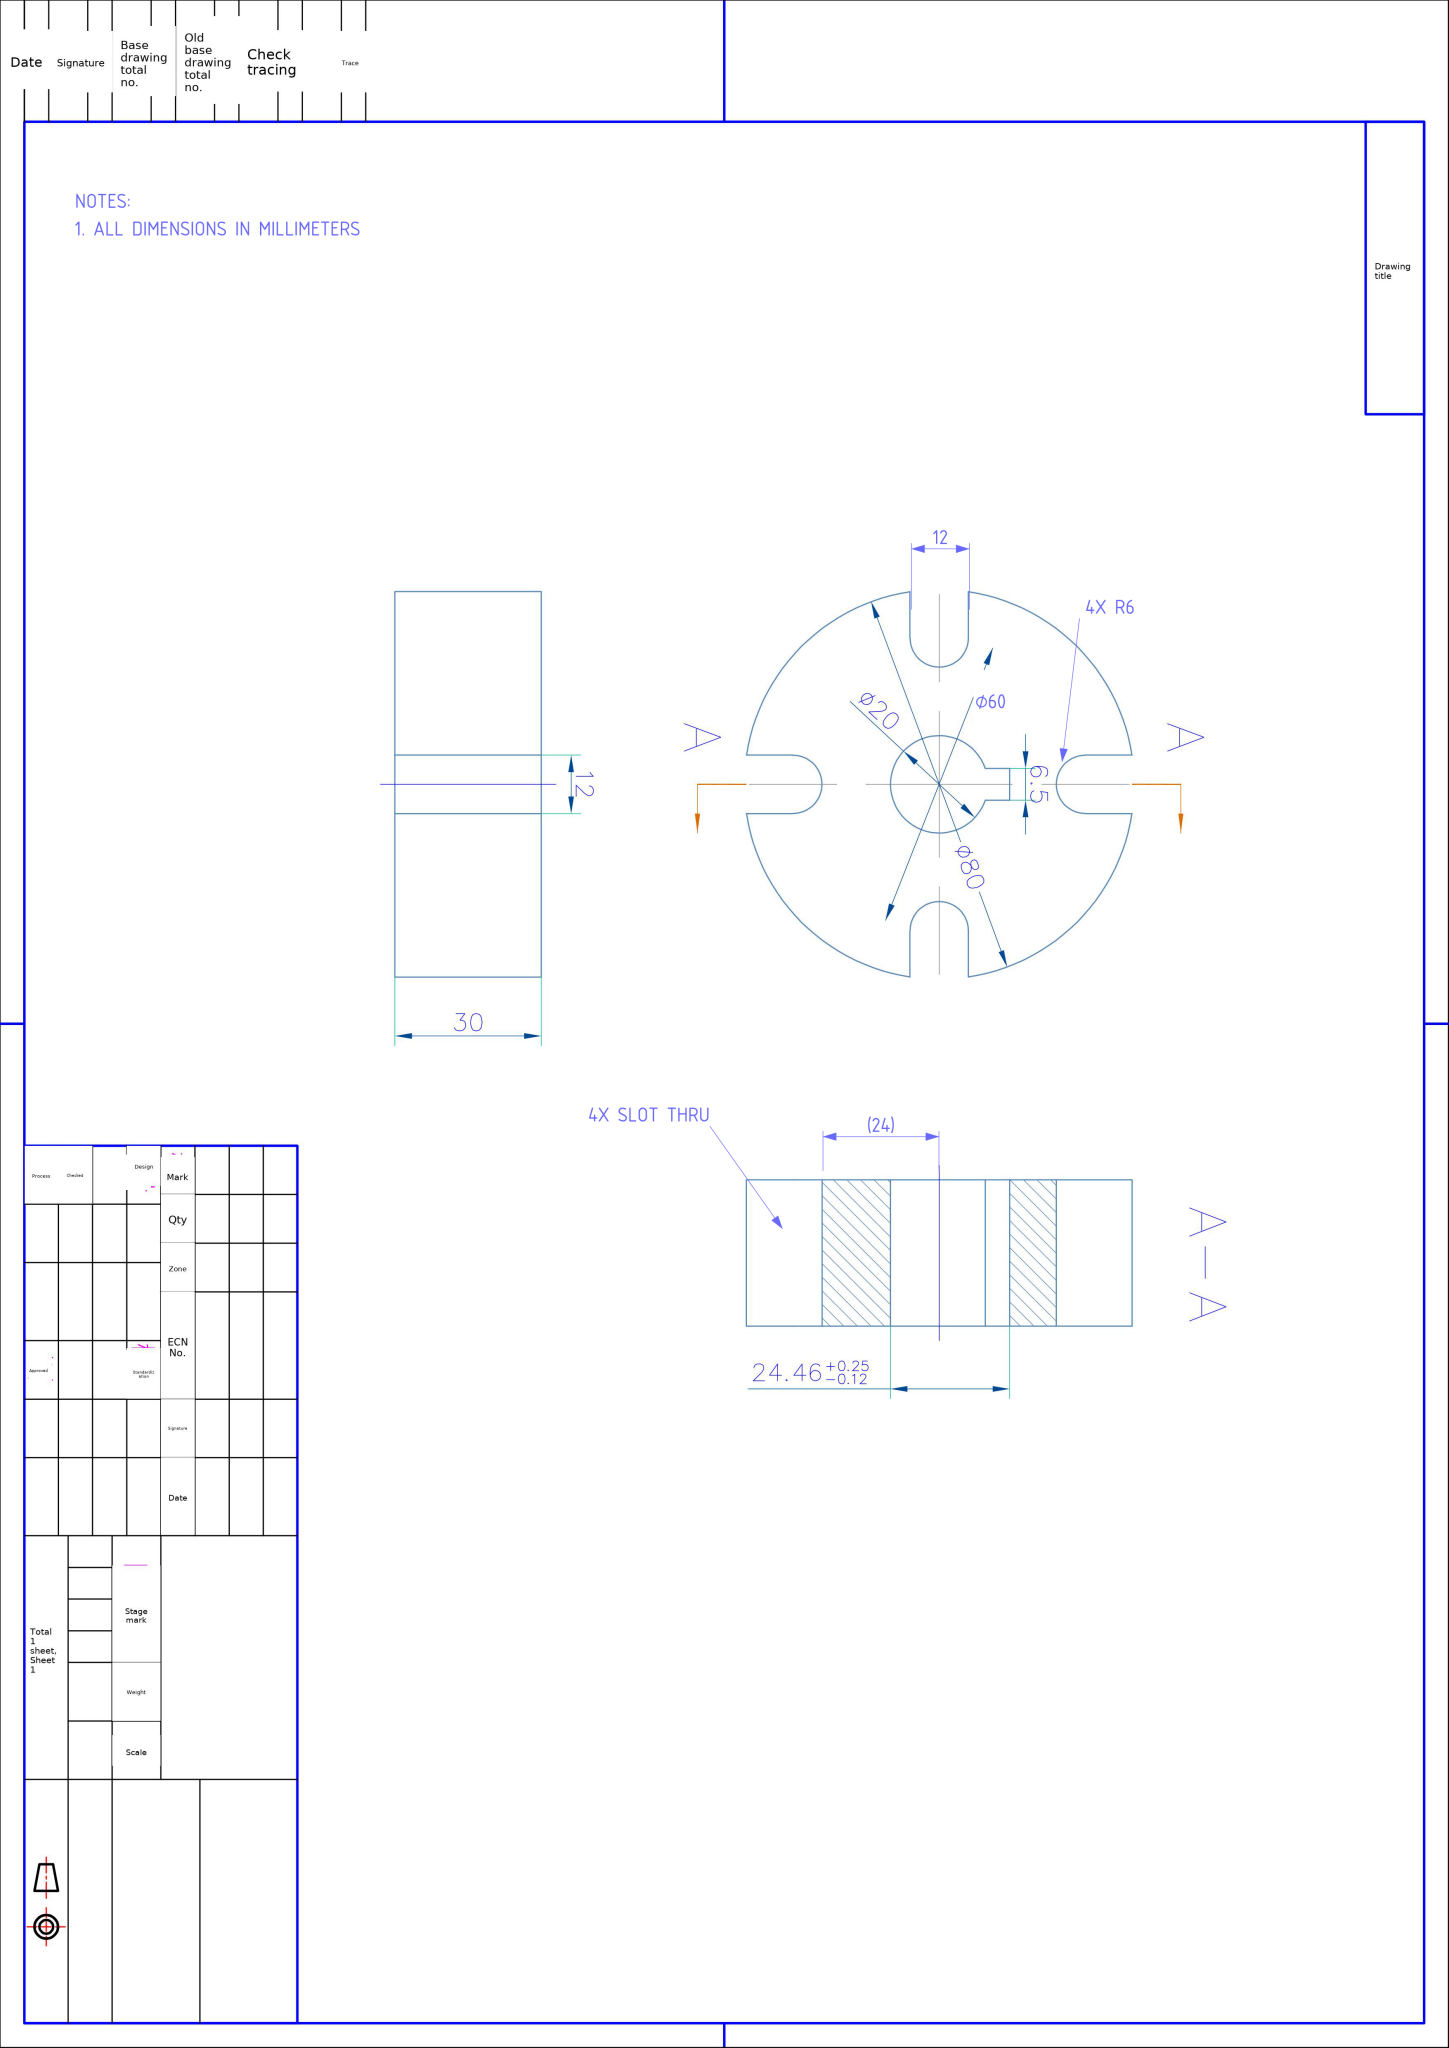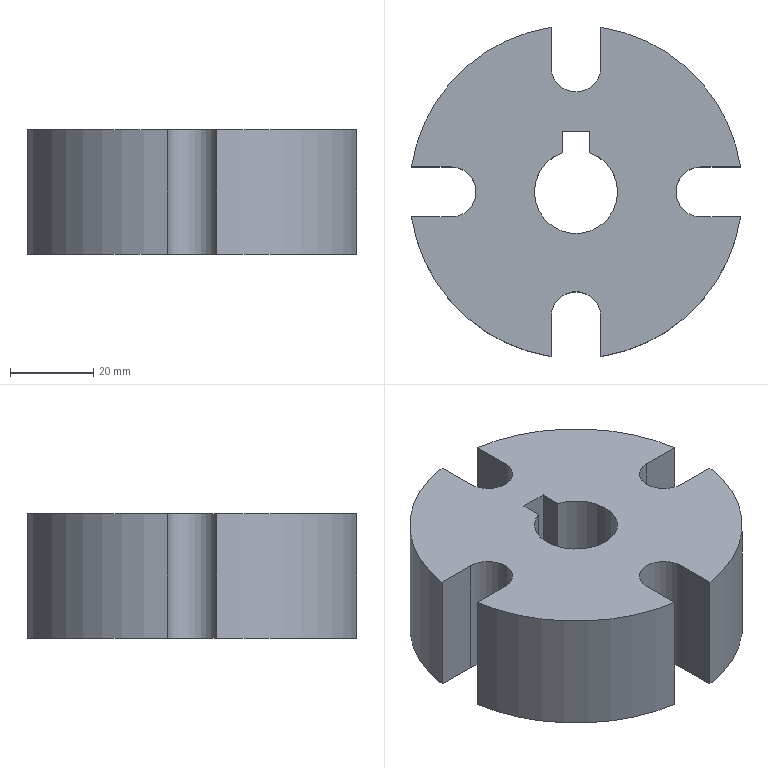Part | NX | mm | 1 solid | 22 faces | box 79.09 x 79.09 x 30 mm | volume 119499 mm3 | plane 13 | cylinder 9 | commonest cylinder face diameters 80 x4 12 x4 20 x1
STEP:
#1=CARTESIAN_POINT('',(0.,0.,0.));
#2=DIRECTION('',(0.,0.,1.));
#3=DIRECTION('',(1.,0.,0.));
#4=AXIS2_PLACEMENT_3D('',#1,#2,#3);
#5=(LENGTH_UNIT()NAMED_UNIT(*)SI_UNIT(.MILLI.,.METRE.));
#6=UNCERTAINTY_MEASURE_WITH_UNIT(LENGTH_MEASURE(0.00002),#5,'','');
#7=(NAMED_UNIT(*)PLANE_ANGLE_UNIT()SI_UNIT($,.RADIAN.));
#8=PLANE_ANGLE_MEASURE_WITH_UNIT(PLANE_ANGLE_MEASURE(0.01745),#7);
#9=DIMENSIONAL_EXPONENTS(0.,0.,0.,0.,0.,0.,0.);
#10=(CONVERSION_BASED_UNIT('',#8)NAMED_UNIT(#9)PLANE_ANGLE_UNIT());
#11=(NAMED_UNIT(*)SI_UNIT($,.STERADIAN.)SOLID_ANGLE_UNIT());
#12=(GEOMETRIC_REPRESENTATION_CONTEXT(3)GLOBAL_UNCERTAINTY_ASSIGNED_CONTEXT((#6))GLOBAL_UNIT_ASSIGNED_CONTEXT((#5,#10,#11))REPRESENTATION_CONTEXT('',''));
#13=SHAPE_REPRESENTATION('',(#4),#12);
#14=CARTESIAN_POINT('',(-3.25,9.457,0.));
#15=VERTEX_POINT('',#14);
#16=CARTESIAN_POINT('',(-3.25,14.457,0.));
#17=VERTEX_POINT('',#16);
#18=CARTESIAN_POINT('',(-3.25,9.457,0.));
#19=DIRECTION('',(0.,1.,0.));
#20=VECTOR('',#19,1.);
#21=LINE('',#18,#20);
#22=EDGE_CURVE('',#15,#17,#21,.T.);
#23=ORIENTED_EDGE('',*,*,#22,.T.);
#24=CARTESIAN_POINT('',(-3.25,14.457,30.));
#25=VERTEX_POINT('',#24);
#26=CARTESIAN_POINT('',(-3.25,14.457,30.));
#27=DIRECTION('',(0.,0.,-1.));
#28=VECTOR('',#27,1.);
#29=LINE('',#26,#28);
#30=EDGE_CURVE('',#25,#17,#29,.T.);
#31=ORIENTED_EDGE('',*,*,#30,.F.);
#32=CARTESIAN_POINT('',(-3.25,9.457,30.));
#33=VERTEX_POINT('',#32);
#34=CARTESIAN_POINT('',(-3.25,9.457,30.));
#35=DIRECTION('',(0.,1.,0.));
#36=VECTOR('',#35,1.);
#37=LINE('',#34,#36);
#38=EDGE_CURVE('',#33,#25,#37,.T.);
#39=ORIENTED_EDGE('',*,*,#38,.F.);
#40=CARTESIAN_POINT('',(-3.25,9.457,30.));
#41=DIRECTION('',(0.,0.,-1.));
#42=VECTOR('',#41,1.);
#43=LINE('',#40,#42);
#44=EDGE_CURVE('',#33,#15,#43,.T.);
#45=ORIENTED_EDGE('',*,*,#44,.T.);
#46=EDGE_LOOP('',(#23,#31,#39,#45));
#47=FACE_OUTER_BOUND('',#46,.T.);
#48=CARTESIAN_POINT('',(-3.25,9.457,30.));
#49=DIRECTION('',(-1.,0.,0.));
#50=DIRECTION('',(0.,0.,1.));
#51=AXIS2_PLACEMENT_3D('',#48,#49,#50);
#52=PLANE('',#51);
#53=ADVANCED_FACE('',(#47),#52,.F.);
#54=CARTESIAN_POINT('',(3.25,14.457,0.));
#55=VERTEX_POINT('',#54);
#56=CARTESIAN_POINT('',(-3.25,14.457,0.));
#57=DIRECTION('',(1.,0.,0.));
#58=VECTOR('',#57,1.);
#59=LINE('',#56,#58);
#60=EDGE_CURVE('',#17,#55,#59,.T.);
#61=ORIENTED_EDGE('',*,*,#60,.T.);
#62=CARTESIAN_POINT('',(3.25,14.457,30.));
#63=VERTEX_POINT('',#62);
#64=CARTESIAN_POINT('',(3.25,14.457,30.));
#65=DIRECTION('',(0.,0.,-1.));
#66=VECTOR('',#65,1.);
#67=LINE('',#64,#66);
#68=EDGE_CURVE('',#63,#55,#67,.T.);
#69=ORIENTED_EDGE('',*,*,#68,.F.);
#70=CARTESIAN_POINT('',(-3.25,14.457,30.));
#71=DIRECTION('',(1.,0.,0.));
#72=VECTOR('',#71,1.);
#73=LINE('',#70,#72);
#74=EDGE_CURVE('',#25,#63,#73,.T.);
#75=ORIENTED_EDGE('',*,*,#74,.F.);
#76=ORIENTED_EDGE('',*,*,#30,.T.);
#77=EDGE_LOOP('',(#61,#69,#75,#76));
#78=FACE_OUTER_BOUND('',#77,.T.);
#79=CARTESIAN_POINT('',(-3.25,14.457,30.));
#80=DIRECTION('',(0.,1.,0.));
#81=DIRECTION('',(0.,0.,1.));
#82=AXIS2_PLACEMENT_3D('',#79,#80,#81);
#83=PLANE('',#82);
#84=ADVANCED_FACE('',(#78),#83,.F.);
#85=CARTESIAN_POINT('',(3.25,9.457,0.));
#86=VERTEX_POINT('',#85);
#87=CARTESIAN_POINT('',(3.25,14.457,0.));
#88=DIRECTION('',(0.,-1.,0.));
#89=VECTOR('',#88,1.);
#90=LINE('',#87,#89);
#91=EDGE_CURVE('',#55,#86,#90,.T.);
#92=ORIENTED_EDGE('',*,*,#91,.T.);
#93=CARTESIAN_POINT('',(3.25,9.457,30.));
#94=VERTEX_POINT('',#93);
#95=CARTESIAN_POINT('',(3.25,9.457,30.));
#96=DIRECTION('',(0.,0.,-1.));
#97=VECTOR('',#96,1.);
#98=LINE('',#95,#97);
#99=EDGE_CURVE('',#94,#86,#98,.T.);
#100=ORIENTED_EDGE('',*,*,#99,.F.);
#101=CARTESIAN_POINT('',(3.25,14.457,30.));
#102=DIRECTION('',(0.,-1.,0.));
#103=VECTOR('',#102,1.);
#104=LINE('',#101,#103);
#105=EDGE_CURVE('',#63,#94,#104,.T.);
#106=ORIENTED_EDGE('',*,*,#105,.F.);
#107=ORIENTED_EDGE('',*,*,#68,.T.);
#108=EDGE_LOOP('',(#92,#100,#106,#107));
#109=FACE_OUTER_BOUND('',#108,.T.);
#110=CARTESIAN_POINT('',(3.25,14.457,30.));
#111=DIRECTION('',(1.,0.,0.));
#112=DIRECTION('',(0.,0.,-1.));
#113=AXIS2_PLACEMENT_3D('',#110,#111,#112);
#114=PLANE('',#113);
#115=ADVANCED_FACE('',(#109),#114,.F.);
#116=CARTESIAN_POINT('',(-30.,-6.,0.));
#117=VERTEX_POINT('',#116);
#118=CARTESIAN_POINT('',(-39.547,-6.,0.));
#119=VERTEX_POINT('',#118);
#120=CARTESIAN_POINT('',(-30.,-6.,0.));
#121=DIRECTION('',(-1.,0.,0.));
#122=VECTOR('',#121,1.);
#123=LINE('',#120,#122);
#124=EDGE_CURVE('',#117,#119,#123,.T.);
#125=ORIENTED_EDGE('',*,*,#124,.T.);
#126=CARTESIAN_POINT('',(-39.547,-6.,30.));
#127=VERTEX_POINT('',#126);
#128=CARTESIAN_POINT('',(-39.547,-6.,30.));
#129=DIRECTION('',(0.,0.,-1.));
#130=VECTOR('',#129,1.);
#131=LINE('',#128,#130);
#132=EDGE_CURVE('',#127,#119,#131,.T.);
#133=ORIENTED_EDGE('',*,*,#132,.F.);
#134=CARTESIAN_POINT('',(-30.,-6.,30.));
#135=VERTEX_POINT('',#134);
#136=CARTESIAN_POINT('',(-30.,-6.,30.));
#137=DIRECTION('',(-1.,0.,0.));
#138=VECTOR('',#137,1.);
#139=LINE('',#136,#138);
#140=EDGE_CURVE('',#135,#127,#139,.T.);
#141=ORIENTED_EDGE('',*,*,#140,.F.);
#142=CARTESIAN_POINT('',(-30.,-6.,30.));
#143=DIRECTION('',(0.,0.,-1.));
#144=VECTOR('',#143,1.);
#145=LINE('',#142,#144);
#146=EDGE_CURVE('',#135,#117,#145,.T.);
#147=ORIENTED_EDGE('',*,*,#146,.T.);
#148=EDGE_LOOP('',(#125,#133,#141,#147));
#149=FACE_OUTER_BOUND('',#148,.T.);
#150=CARTESIAN_POINT('',(-30.,-6.,30.));
#151=DIRECTION('',(-0.,-1.,0.));
#152=DIRECTION('',(1.,-0.,0.));
#153=AXIS2_PLACEMENT_3D('',#150,#151,#152);
#154=PLANE('',#153);
#155=ADVANCED_FACE('',(#149),#154,.F.);
#156=CARTESIAN_POINT('',(-6.,-39.547,0.));
#157=VERTEX_POINT('',#156);
#158=CARTESIAN_POINT('',(0.,0.,0.));
#159=DIRECTION('',(0.,0.,1.));
#160=DIRECTION('',(1.,0.,0.));
#161=AXIS2_PLACEMENT_3D('',#158,#159,#160);
#162=CIRCLE('',#161,40.);
#163=EDGE_CURVE('',#119,#157,#162,.T.);
#164=ORIENTED_EDGE('',*,*,#163,.T.);
#165=CARTESIAN_POINT('',(-6.,-39.547,30.));
#166=VERTEX_POINT('',#165);
#167=CARTESIAN_POINT('',(-6.,-39.547,30.));
#168=DIRECTION('',(0.,0.,-1.));
#169=VECTOR('',#168,1.);
#170=LINE('',#167,#169);
#171=EDGE_CURVE('',#166,#157,#170,.T.);
#172=ORIENTED_EDGE('',*,*,#171,.F.);
#173=CARTESIAN_POINT('',(0.,0.,30.));
#174=DIRECTION('',(0.,0.,1.));
#175=DIRECTION('',(1.,0.,0.));
#176=AXIS2_PLACEMENT_3D('',#173,#174,#175);
#177=CIRCLE('',#176,40.);
#178=EDGE_CURVE('',#127,#166,#177,.T.);
#179=ORIENTED_EDGE('',*,*,#178,.F.);
#180=ORIENTED_EDGE('',*,*,#132,.T.);
#181=EDGE_LOOP('',(#164,#172,#179,#180));
#182=FACE_OUTER_BOUND('',#181,.T.);
#183=CARTESIAN_POINT('',(0.,0.,30.));
#184=DIRECTION('',(0.,0.,-1.));
#185=DIRECTION('',(-1.,0.,0.));
#186=AXIS2_PLACEMENT_3D('',#183,#184,#185);
#187=CYLINDRICAL_SURFACE('',#186,40.);
#188=ADVANCED_FACE('',(#182),#187,.T.);
#189=CARTESIAN_POINT('',(-6.,-30.,0.));
#190=VERTEX_POINT('',#189);
#191=CARTESIAN_POINT('',(-6.,-39.547,0.));
#192=DIRECTION('',(0.,1.,0.));
#193=VECTOR('',#192,1.);
#194=LINE('',#191,#193);
#195=EDGE_CURVE('',#157,#190,#194,.T.);
#196=ORIENTED_EDGE('',*,*,#195,.T.);
#197=CARTESIAN_POINT('',(-6.,-30.,30.));
#198=VERTEX_POINT('',#197);
#199=CARTESIAN_POINT('',(-6.,-30.,30.));
#200=DIRECTION('',(0.,0.,-1.));
#201=VECTOR('',#200,1.);
#202=LINE('',#199,#201);
#203=EDGE_CURVE('',#198,#190,#202,.T.);
#204=ORIENTED_EDGE('',*,*,#203,.F.);
#205=CARTESIAN_POINT('',(-6.,-39.547,30.));
#206=DIRECTION('',(0.,1.,0.));
#207=VECTOR('',#206,1.);
#208=LINE('',#205,#207);
#209=EDGE_CURVE('',#166,#198,#208,.T.);
#210=ORIENTED_EDGE('',*,*,#209,.F.);
#211=ORIENTED_EDGE('',*,*,#171,.T.);
#212=EDGE_LOOP('',(#196,#204,#210,#211));
#213=FACE_OUTER_BOUND('',#212,.T.);
#214=CARTESIAN_POINT('',(-6.,-39.547,30.));
#215=DIRECTION('',(-1.,0.,0.));
#216=DIRECTION('',(-0.,-1.,0.));
#217=AXIS2_PLACEMENT_3D('',#214,#215,#216);
#218=PLANE('',#217);
#219=ADVANCED_FACE('',(#213),#218,.F.);
#220=CARTESIAN_POINT('',(6.,-30.,0.));
#221=VERTEX_POINT('',#220);
#222=CARTESIAN_POINT('',(0.,-30.,0.));
#223=DIRECTION('',(0.,0.,-1.));
#224=DIRECTION('',(1.,0.,0.));
#225=AXIS2_PLACEMENT_3D('',#222,#223,#224);
#226=CIRCLE('',#225,6.);
#227=EDGE_CURVE('',#190,#221,#226,.T.);
#228=ORIENTED_EDGE('',*,*,#227,.T.);
#229=CARTESIAN_POINT('',(6.,-30.,30.));
#230=VERTEX_POINT('',#229);
#231=CARTESIAN_POINT('',(6.,-30.,30.));
#232=DIRECTION('',(0.,0.,-1.));
#233=VECTOR('',#232,1.);
#234=LINE('',#231,#233);
#235=EDGE_CURVE('',#230,#221,#234,.T.);
#236=ORIENTED_EDGE('',*,*,#235,.F.);
#237=CARTESIAN_POINT('',(0.,-30.,30.));
#238=DIRECTION('',(0.,0.,-1.));
#239=DIRECTION('',(1.,0.,0.));
#240=AXIS2_PLACEMENT_3D('',#237,#238,#239);
#241=CIRCLE('',#240,6.);
#242=EDGE_CURVE('',#198,#230,#241,.T.);
#243=ORIENTED_EDGE('',*,*,#242,.F.);
#244=ORIENTED_EDGE('',*,*,#203,.T.);
#245=EDGE_LOOP('',(#228,#236,#243,#244));
#246=FACE_OUTER_BOUND('',#245,.T.);
#247=CARTESIAN_POINT('',(0.,-30.,30.));
#248=DIRECTION('',(0.,0.,-1.));
#249=DIRECTION('',(-1.,0.,0.));
#250=AXIS2_PLACEMENT_3D('',#247,#248,#249);
#251=CYLINDRICAL_SURFACE('',#250,6.);
#252=ADVANCED_FACE('',(#246),#251,.F.);
#253=CARTESIAN_POINT('',(6.,-39.547,0.));
#254=VERTEX_POINT('',#253);
#255=CARTESIAN_POINT('',(6.,-30.,0.));
#256=DIRECTION('',(0.,-1.,0.));
#257=VECTOR('',#256,1.);
#258=LINE('',#255,#257);
#259=EDGE_CURVE('',#221,#254,#258,.T.);
#260=ORIENTED_EDGE('',*,*,#259,.T.);
#261=CARTESIAN_POINT('',(6.,-39.547,30.));
#262=VERTEX_POINT('',#261);
#263=CARTESIAN_POINT('',(6.,-39.547,30.));
#264=DIRECTION('',(0.,0.,-1.));
#265=VECTOR('',#264,1.);
#266=LINE('',#263,#265);
#267=EDGE_CURVE('',#262,#254,#266,.T.);
#268=ORIENTED_EDGE('',*,*,#267,.F.);
#269=CARTESIAN_POINT('',(6.,-30.,30.));
#270=DIRECTION('',(0.,-1.,0.));
#271=VECTOR('',#270,1.);
#272=LINE('',#269,#271);
#273=EDGE_CURVE('',#230,#262,#272,.T.);
#274=ORIENTED_EDGE('',*,*,#273,.F.);
#275=ORIENTED_EDGE('',*,*,#235,.T.);
#276=EDGE_LOOP('',(#260,#268,#274,#275));
#277=FACE_OUTER_BOUND('',#276,.T.);
#278=CARTESIAN_POINT('',(6.,-30.,30.));
#279=DIRECTION('',(1.,0.,0.));
#280=DIRECTION('',(-0.,1.,0.));
#281=AXIS2_PLACEMENT_3D('',#278,#279,#280);
#282=PLANE('',#281);
#283=ADVANCED_FACE('',(#277),#282,.F.);
#284=CARTESIAN_POINT('',(39.547,-6.,0.));
#285=VERTEX_POINT('',#284);
#286=CARTESIAN_POINT('',(0.,0.,0.));
#287=DIRECTION('',(0.,0.,1.));
#288=DIRECTION('',(1.,0.,0.));
#289=AXIS2_PLACEMENT_3D('',#286,#287,#288);
#290=CIRCLE('',#289,40.);
#291=EDGE_CURVE('',#254,#285,#290,.T.);
#292=ORIENTED_EDGE('',*,*,#291,.T.);
#293=CARTESIAN_POINT('',(39.547,-6.,30.));
#294=VERTEX_POINT('',#293);
#295=CARTESIAN_POINT('',(39.547,-6.,30.));
#296=DIRECTION('',(0.,0.,-1.));
#297=VECTOR('',#296,1.);
#298=LINE('',#295,#297);
#299=EDGE_CURVE('',#294,#285,#298,.T.);
#300=ORIENTED_EDGE('',*,*,#299,.F.);
#301=CARTESIAN_POINT('',(0.,0.,30.));
#302=DIRECTION('',(0.,0.,1.));
#303=DIRECTION('',(1.,0.,0.));
#304=AXIS2_PLACEMENT_3D('',#301,#302,#303);
#305=CIRCLE('',#304,40.);
#306=EDGE_CURVE('',#262,#294,#305,.T.);
#307=ORIENTED_EDGE('',*,*,#306,.F.);
#308=ORIENTED_EDGE('',*,*,#267,.T.);
#309=EDGE_LOOP('',(#292,#300,#307,#308));
#310=FACE_OUTER_BOUND('',#309,.T.);
#311=CARTESIAN_POINT('',(0.,0.,30.));
#312=DIRECTION('',(0.,0.,-1.));
#313=DIRECTION('',(-1.,0.,0.));
#314=AXIS2_PLACEMENT_3D('',#311,#312,#313);
#315=CYLINDRICAL_SURFACE('',#314,40.);
#316=ADVANCED_FACE('',(#310),#315,.T.);
#317=CARTESIAN_POINT('',(30.,-6.,0.));
#318=VERTEX_POINT('',#317);
#319=CARTESIAN_POINT('',(39.547,-6.,0.));
#320=DIRECTION('',(-1.,-0.,0.));
#321=VECTOR('',#320,1.);
#322=LINE('',#319,#321);
#323=EDGE_CURVE('',#285,#318,#322,.T.);
#324=ORIENTED_EDGE('',*,*,#323,.T.);
#325=CARTESIAN_POINT('',(30.,-6.,30.));
#326=VERTEX_POINT('',#325);
#327=CARTESIAN_POINT('',(30.,-6.,30.));
#328=DIRECTION('',(0.,0.,-1.));
#329=VECTOR('',#328,1.);
#330=LINE('',#327,#329);
#331=EDGE_CURVE('',#326,#318,#330,.T.);
#332=ORIENTED_EDGE('',*,*,#331,.F.);
#333=CARTESIAN_POINT('',(39.547,-6.,30.));
#334=DIRECTION('',(-1.,-0.,0.));
#335=VECTOR('',#334,1.);
#336=LINE('',#333,#335);
#337=EDGE_CURVE('',#294,#326,#336,.T.);
#338=ORIENTED_EDGE('',*,*,#337,.F.);
#339=ORIENTED_EDGE('',*,*,#299,.T.);
#340=EDGE_LOOP('',(#324,#332,#338,#339));
#341=FACE_OUTER_BOUND('',#340,.T.);
#342=CARTESIAN_POINT('',(39.547,-6.,30.));
#343=DIRECTION('',(0.,-1.,0.));
#344=DIRECTION('',(1.,0.,0.));
#345=AXIS2_PLACEMENT_3D('',#342,#343,#344);
#346=PLANE('',#345);
#347=ADVANCED_FACE('',(#341),#346,.F.);
#348=CARTESIAN_POINT('',(30.,6.,0.));
#349=VERTEX_POINT('',#348);
#350=CARTESIAN_POINT('',(30.,0.,0.));
#351=DIRECTION('',(0.,0.,-1.));
#352=DIRECTION('',(1.,0.,0.));
#353=AXIS2_PLACEMENT_3D('',#350,#351,#352);
#354=CIRCLE('',#353,6.);
#355=EDGE_CURVE('',#318,#349,#354,.T.);
#356=ORIENTED_EDGE('',*,*,#355,.T.);
#357=CARTESIAN_POINT('',(30.,6.,30.));
#358=VERTEX_POINT('',#357);
#359=CARTESIAN_POINT('',(30.,6.,30.));
#360=DIRECTION('',(0.,0.,-1.));
#361=VECTOR('',#360,1.);
#362=LINE('',#359,#361);
#363=EDGE_CURVE('',#358,#349,#362,.T.);
#364=ORIENTED_EDGE('',*,*,#363,.F.);
#365=CARTESIAN_POINT('',(30.,0.,30.));
#366=DIRECTION('',(0.,0.,-1.));
#367=DIRECTION('',(1.,0.,0.));
#368=AXIS2_PLACEMENT_3D('',#365,#366,#367);
#369=CIRCLE('',#368,6.);
#370=EDGE_CURVE('',#326,#358,#369,.T.);
#371=ORIENTED_EDGE('',*,*,#370,.F.);
#372=ORIENTED_EDGE('',*,*,#331,.T.);
#373=EDGE_LOOP('',(#356,#364,#371,#372));
#374=FACE_OUTER_BOUND('',#373,.T.);
#375=CARTESIAN_POINT('',(30.,0.,30.));
#376=DIRECTION('',(0.,0.,-1.));
#377=DIRECTION('',(-1.,0.,0.));
#378=AXIS2_PLACEMENT_3D('',#375,#376,#377);
#379=CYLINDRICAL_SURFACE('',#378,6.);
#380=ADVANCED_FACE('',(#374),#379,.F.);
#381=CARTESIAN_POINT('',(39.547,6.,0.));
#382=VERTEX_POINT('',#381);
#383=CARTESIAN_POINT('',(30.,6.,0.));
#384=DIRECTION('',(1.,-0.,0.));
#385=VECTOR('',#384,1.);
#386=LINE('',#383,#385);
#387=EDGE_CURVE('',#349,#382,#386,.T.);
#388=ORIENTED_EDGE('',*,*,#387,.T.);
#389=CARTESIAN_POINT('',(39.547,6.,30.));
#390=VERTEX_POINT('',#389);
#391=CARTESIAN_POINT('',(39.547,6.,30.));
#392=DIRECTION('',(0.,0.,-1.));
#393=VECTOR('',#392,1.);
#394=LINE('',#391,#393);
#395=EDGE_CURVE('',#390,#382,#394,.T.);
#396=ORIENTED_EDGE('',*,*,#395,.F.);
#397=CARTESIAN_POINT('',(30.,6.,30.));
#398=DIRECTION('',(1.,-0.,0.));
#399=VECTOR('',#398,1.);
#400=LINE('',#397,#399);
#401=EDGE_CURVE('',#358,#390,#400,.T.);
#402=ORIENTED_EDGE('',*,*,#401,.F.);
#403=ORIENTED_EDGE('',*,*,#363,.T.);
#404=EDGE_LOOP('',(#388,#396,#402,#403));
#405=FACE_OUTER_BOUND('',#404,.T.);
#406=CARTESIAN_POINT('',(30.,6.,30.));
#407=DIRECTION('',(0.,1.,0.));
#408=DIRECTION('',(-1.,0.,0.));
#409=AXIS2_PLACEMENT_3D('',#406,#407,#408);
#410=PLANE('',#409);
#411=ADVANCED_FACE('',(#405),#410,.F.);
#412=CARTESIAN_POINT('',(6.,39.547,0.));
#413=VERTEX_POINT('',#412);
#414=CARTESIAN_POINT('',(0.,0.,0.));
#415=DIRECTION('',(0.,0.,1.));
#416=DIRECTION('',(1.,0.,0.));
#417=AXIS2_PLACEMENT_3D('',#414,#415,#416);
#418=CIRCLE('',#417,40.);
#419=EDGE_CURVE('',#382,#413,#418,.T.);
#420=ORIENTED_EDGE('',*,*,#419,.T.);
#421=CARTESIAN_POINT('',(6.,39.547,30.));
#422=VERTEX_POINT('',#421);
#423=CARTESIAN_POINT('',(6.,39.547,30.));
#424=DIRECTION('',(0.,0.,-1.));
#425=VECTOR('',#424,1.);
#426=LINE('',#423,#425);
#427=EDGE_CURVE('',#422,#413,#426,.T.);
#428=ORIENTED_EDGE('',*,*,#427,.F.);
#429=CARTESIAN_POINT('',(0.,0.,30.));
#430=DIRECTION('',(0.,0.,1.));
#431=DIRECTION('',(1.,0.,0.));
#432=AXIS2_PLACEMENT_3D('',#429,#430,#431);
#433=CIRCLE('',#432,40.);
#434=EDGE_CURVE('',#390,#422,#433,.T.);
#435=ORIENTED_EDGE('',*,*,#434,.F.);
#436=ORIENTED_EDGE('',*,*,#395,.T.);
#437=EDGE_LOOP('',(#420,#428,#435,#436));
#438=FACE_OUTER_BOUND('',#437,.T.);
#439=CARTESIAN_POINT('',(0.,0.,30.));
#440=DIRECTION('',(0.,0.,-1.));
#441=DIRECTION('',(-1.,0.,0.));
#442=AXIS2_PLACEMENT_3D('',#439,#440,#441);
#443=CYLINDRICAL_SURFACE('',#442,40.);
#444=ADVANCED_FACE('',(#438),#443,.T.);
#445=CARTESIAN_POINT('',(6.,30.,0.));
#446=VERTEX_POINT('',#445);
#447=CARTESIAN_POINT('',(6.,39.547,0.));
#448=DIRECTION('',(-0.,-1.,0.));
#449=VECTOR('',#448,1.);
#450=LINE('',#447,#449);
#451=EDGE_CURVE('',#413,#446,#450,.T.);
#452=ORIENTED_EDGE('',*,*,#451,.T.);
#453=CARTESIAN_POINT('',(6.,30.,30.));
#454=VERTEX_POINT('',#453);
#455=CARTESIAN_POINT('',(6.,30.,30.));
#456=DIRECTION('',(0.,0.,-1.));
#457=VECTOR('',#456,1.);
#458=LINE('',#455,#457);
#459=EDGE_CURVE('',#454,#446,#458,.T.);
#460=ORIENTED_EDGE('',*,*,#459,.F.);
#461=CARTESIAN_POINT('',(6.,39.547,30.));
#462=DIRECTION('',(-0.,-1.,0.));
#463=VECTOR('',#462,1.);
#464=LINE('',#461,#463);
#465=EDGE_CURVE('',#422,#454,#464,.T.);
#466=ORIENTED_EDGE('',*,*,#465,.F.);
#467=ORIENTED_EDGE('',*,*,#427,.T.);
#468=EDGE_LOOP('',(#452,#460,#466,#467));
#469=FACE_OUTER_BOUND('',#468,.T.);
#470=CARTESIAN_POINT('',(6.,39.547,30.));
#471=DIRECTION('',(1.,-0.,0.));
#472=DIRECTION('',(0.,1.,0.));
#473=AXIS2_PLACEMENT_3D('',#470,#471,#472);
#474=PLANE('',#473);
#475=ADVANCED_FACE('',(#469),#474,.F.);
#476=CARTESIAN_POINT('',(-6.,30.,0.));
#477=VERTEX_POINT('',#476);
#478=CARTESIAN_POINT('',(0.,30.,0.));
#479=DIRECTION('',(0.,0.,-1.));
#480=DIRECTION('',(1.,0.,0.));
#481=AXIS2_PLACEMENT_3D('',#478,#479,#480);
#482=CIRCLE('',#481,6.);
#483=EDGE_CURVE('',#446,#477,#482,.T.);
#484=ORIENTED_EDGE('',*,*,#483,.T.);
#485=CARTESIAN_POINT('',(-6.,30.,30.));
#486=VERTEX_POINT('',#485);
#487=CARTESIAN_POINT('',(-6.,30.,30.));
#488=DIRECTION('',(0.,0.,-1.));
#489=VECTOR('',#488,1.);
#490=LINE('',#487,#489);
#491=EDGE_CURVE('',#486,#477,#490,.T.);
#492=ORIENTED_EDGE('',*,*,#491,.F.);
#493=CARTESIAN_POINT('',(0.,30.,30.));
#494=DIRECTION('',(0.,0.,-1.));
#495=DIRECTION('',(1.,0.,0.));
#496=AXIS2_PLACEMENT_3D('',#493,#494,#495);
#497=CIRCLE('',#496,6.);
#498=EDGE_CURVE('',#454,#486,#497,.T.);
#499=ORIENTED_EDGE('',*,*,#498,.F.);
#500=ORIENTED_EDGE('',*,*,#459,.T.);
#501=EDGE_LOOP('',(#484,#492,#499,#500));
#502=FACE_OUTER_BOUND('',#501,.T.);
#503=CARTESIAN_POINT('',(0.,30.,30.));
#504=DIRECTION('',(0.,0.,-1.));
#505=DIRECTION('',(-1.,0.,0.));
#506=AXIS2_PLACEMENT_3D('',#503,#504,#505);
#507=CYLINDRICAL_SURFACE('',#506,6.);
#508=ADVANCED_FACE('',(#502),#507,.F.);
#509=CARTESIAN_POINT('',(-6.,39.547,0.));
#510=VERTEX_POINT('',#509);
#511=CARTESIAN_POINT('',(-6.,30.,0.));
#512=DIRECTION('',(-0.,1.,0.));
#513=VECTOR('',#512,1.);
#514=LINE('',#511,#513);
#515=EDGE_CURVE('',#477,#510,#514,.T.);
#516=ORIENTED_EDGE('',*,*,#515,.T.);
#517=CARTESIAN_POINT('',(-6.,39.547,30.));
#518=VERTEX_POINT('',#517);
#519=CARTESIAN_POINT('',(-6.,39.547,30.));
#520=DIRECTION('',(0.,0.,-1.));
#521=VECTOR('',#520,1.);
#522=LINE('',#519,#521);
#523=EDGE_CURVE('',#518,#510,#522,.T.);
#524=ORIENTED_EDGE('',*,*,#523,.F.);
#525=CARTESIAN_POINT('',(-6.,30.,30.));
#526=DIRECTION('',(-0.,1.,0.));
#527=VECTOR('',#526,1.);
#528=LINE('',#525,#527);
#529=EDGE_CURVE('',#486,#518,#528,.T.);
#530=ORIENTED_EDGE('',*,*,#529,.F.);
#531=ORIENTED_EDGE('',*,*,#491,.T.);
#532=EDGE_LOOP('',(#516,#524,#530,#531));
#533=FACE_OUTER_BOUND('',#532,.T.);
#534=CARTESIAN_POINT('',(-6.,30.,30.));
#535=DIRECTION('',(-1.,-0.,0.));
#536=DIRECTION('',(0.,-1.,0.));
#537=AXIS2_PLACEMENT_3D('',#534,#535,#536);
#538=PLANE('',#537);
#539=ADVANCED_FACE('',(#533),#538,.F.);
#540=CARTESIAN_POINT('',(-39.547,6.,0.));
#541=VERTEX_POINT('',#540);
#542=CARTESIAN_POINT('',(0.,0.,0.));
#543=DIRECTION('',(0.,0.,1.));
#544=DIRECTION('',(1.,0.,0.));
#545=AXIS2_PLACEMENT_3D('',#542,#543,#544);
#546=CIRCLE('',#545,40.);
#547=EDGE_CURVE('',#510,#541,#546,.T.);
#548=ORIENTED_EDGE('',*,*,#547,.T.);
#549=CARTESIAN_POINT('',(-39.547,6.,30.));
#550=VERTEX_POINT('',#549);
#551=CARTESIAN_POINT('',(-39.547,6.,30.));
#552=DIRECTION('',(0.,0.,-1.));
#553=VECTOR('',#552,1.);
#554=LINE('',#551,#553);
#555=EDGE_CURVE('',#550,#541,#554,.T.);
#556=ORIENTED_EDGE('',*,*,#555,.F.);
#557=CARTESIAN_POINT('',(0.,0.,30.));
#558=DIRECTION('',(0.,0.,1.));
#559=DIRECTION('',(1.,0.,0.));
#560=AXIS2_PLACEMENT_3D('',#557,#558,#559);
#561=CIRCLE('',#560,40.);
#562=EDGE_CURVE('',#518,#550,#561,.T.);
#563=ORIENTED_EDGE('',*,*,#562,.F.);
#564=ORIENTED_EDGE('',*,*,#523,.T.);
#565=EDGE_LOOP('',(#548,#556,#563,#564));
#566=FACE_OUTER_BOUND('',#565,.T.);
#567=CARTESIAN_POINT('',(0.,0.,30.));
#568=DIRECTION('',(0.,0.,-1.));
#569=DIRECTION('',(-1.,0.,0.));
#570=AXIS2_PLACEMENT_3D('',#567,#568,#569);
#571=CYLINDRICAL_SURFACE('',#570,40.);
#572=ADVANCED_FACE('',(#566),#571,.T.);
#573=CARTESIAN_POINT('',(-30.,6.,0.));
#574=VERTEX_POINT('',#573);
#575=CARTESIAN_POINT('',(-39.547,6.,0.));
#576=DIRECTION('',(1.,0.,0.));
#577=VECTOR('',#576,1.);
#578=LINE('',#575,#577);
#579=EDGE_CURVE('',#541,#574,#578,.T.);
#580=ORIENTED_EDGE('',*,*,#579,.T.);
#581=CARTESIAN_POINT('',(-30.,6.,30.));
#582=VERTEX_POINT('',#581);
#583=CARTESIAN_POINT('',(-30.,6.,30.));
#584=DIRECTION('',(0.,0.,-1.));
#585=VECTOR('',#584,1.);
#586=LINE('',#583,#585);
#587=EDGE_CURVE('',#582,#574,#586,.T.);
#588=ORIENTED_EDGE('',*,*,#587,.F.);
#589=CARTESIAN_POINT('',(-39.547,6.,30.));
#590=DIRECTION('',(1.,0.,0.));
#591=VECTOR('',#590,1.);
#592=LINE('',#589,#591);
#593=EDGE_CURVE('',#550,#582,#592,.T.);
#594=ORIENTED_EDGE('',*,*,#593,.F.);
#595=ORIENTED_EDGE('',*,*,#555,.T.);
#596=EDGE_LOOP('',(#580,#588,#594,#595));
#597=FACE_OUTER_BOUND('',#596,.T.);
#598=CARTESIAN_POINT('',(-39.547,6.,30.));
#599=DIRECTION('',(-0.,1.,0.));
#600=DIRECTION('',(-1.,-0.,0.));
#601=AXIS2_PLACEMENT_3D('',#598,#599,#600);
#602=PLANE('',#601);
#603=ADVANCED_FACE('',(#597),#602,.F.);
#604=CARTESIAN_POINT('',(-30.,0.,0.));
#605=DIRECTION('',(0.,0.,-1.));
#606=DIRECTION('',(1.,0.,0.));
#607=AXIS2_PLACEMENT_3D('',#604,#605,#606);
#608=CIRCLE('',#607,6.);
#609=EDGE_CURVE('',#574,#117,#608,.T.);
#610=ORIENTED_EDGE('',*,*,#609,.T.);
#611=ORIENTED_EDGE('',*,*,#146,.F.);
#612=CARTESIAN_POINT('',(-30.,0.,30.));
#613=DIRECTION('',(0.,0.,-1.));
#614=DIRECTION('',(1.,0.,0.));
#615=AXIS2_PLACEMENT_3D('',#612,#613,#614);
#616=CIRCLE('',#615,6.);
#617=EDGE_CURVE('',#582,#135,#616,.T.);
#618=ORIENTED_EDGE('',*,*,#617,.F.);
#619=ORIENTED_EDGE('',*,*,#587,.T.);
#620=EDGE_LOOP('',(#610,#611,#618,#619));
#621=FACE_OUTER_BOUND('',#620,.T.);
#622=CARTESIAN_POINT('',(-30.,0.,30.));
#623=DIRECTION('',(0.,0.,-1.));
#624=DIRECTION('',(-1.,0.,0.));
#625=AXIS2_PLACEMENT_3D('',#622,#623,#624);
#626=CYLINDRICAL_SURFACE('',#625,6.);
#627=ADVANCED_FACE('',(#621),#626,.F.);
#628=CARTESIAN_POINT('',(0.,0.,0.));
#629=DIRECTION('',(0.,0.,-1.));
#630=DIRECTION('',(1.,0.,0.));
#631=AXIS2_PLACEMENT_3D('',#628,#629,#630);
#632=CIRCLE('',#631,10.);
#633=EDGE_CURVE('',#86,#15,#632,.T.);
#634=ORIENTED_EDGE('',*,*,#633,.T.);
#635=ORIENTED_EDGE('',*,*,#44,.F.);
#636=CARTESIAN_POINT('',(0.,0.,30.));
#637=DIRECTION('',(0.,0.,-1.));
#638=DIRECTION('',(1.,0.,0.));
#639=AXIS2_PLACEMENT_3D('',#636,#637,#638);
#640=CIRCLE('',#639,10.);
#641=EDGE_CURVE('',#94,#33,#640,.T.);
#642=ORIENTED_EDGE('',*,*,#641,.F.);
#643=ORIENTED_EDGE('',*,*,#99,.T.);
#644=EDGE_LOOP('',(#634,#635,#642,#643));
#645=FACE_OUTER_BOUND('',#644,.T.);
#646=CARTESIAN_POINT('',(0.,0.,30.));
#647=DIRECTION('',(0.,0.,-1.));
#648=DIRECTION('',(-1.,0.,0.));
#649=AXIS2_PLACEMENT_3D('',#646,#647,#648);
#650=CYLINDRICAL_SURFACE('',#649,10.);
#651=ADVANCED_FACE('',(#645),#650,.F.);
#652=ORIENTED_EDGE('',*,*,#140,.T.);
#653=ORIENTED_EDGE('',*,*,#178,.T.);
#654=ORIENTED_EDGE('',*,*,#209,.T.);
#655=ORIENTED_EDGE('',*,*,#242,.T.);
#656=ORIENTED_EDGE('',*,*,#273,.T.);
#657=ORIENTED_EDGE('',*,*,#306,.T.);
#658=ORIENTED_EDGE('',*,*,#337,.T.);
#659=ORIENTED_EDGE('',*,*,#370,.T.);
#660=ORIENTED_EDGE('',*,*,#401,.T.);
#661=ORIENTED_EDGE('',*,*,#434,.T.);
#662=ORIENTED_EDGE('',*,*,#465,.T.);
#663=ORIENTED_EDGE('',*,*,#498,.T.);
#664=ORIENTED_EDGE('',*,*,#529,.T.);
#665=ORIENTED_EDGE('',*,*,#562,.T.);
#666=ORIENTED_EDGE('',*,*,#593,.T.);
#667=ORIENTED_EDGE('',*,*,#617,.T.);
#668=EDGE_LOOP('',(#652,#653,#654,#655,#656,#657,#658,#659,#660,#661,#662,#663,#664,#665,#666,#667));
#669=FACE_BOUND('',#668,.T.);
#670=ORIENTED_EDGE('',*,*,#38,.T.);
#671=ORIENTED_EDGE('',*,*,#74,.T.);
#672=ORIENTED_EDGE('',*,*,#105,.T.);
#673=ORIENTED_EDGE('',*,*,#641,.T.);
#674=EDGE_LOOP('',(#670,#671,#672,#673));
#675=FACE_BOUND('',#674,.T.);
#676=CARTESIAN_POINT('',(0.,0.,30.));
#677=DIRECTION('',(0.,0.,1.));
#678=DIRECTION('',(1.,0.,0.));
#679=AXIS2_PLACEMENT_3D('',#676,#677,#678);
#680=PLANE('',#679);
#681=ADVANCED_FACE('',(#669,#675),#680,.T.);
#682=ORIENTED_EDGE('',*,*,#124,.F.);
#683=ORIENTED_EDGE('',*,*,#609,.F.);
#684=ORIENTED_EDGE('',*,*,#579,.F.);
#685=ORIENTED_EDGE('',*,*,#547,.F.);
#686=ORIENTED_EDGE('',*,*,#515,.F.);
#687=ORIENTED_EDGE('',*,*,#483,.F.);
#688=ORIENTED_EDGE('',*,*,#451,.F.);
#689=ORIENTED_EDGE('',*,*,#419,.F.);
#690=ORIENTED_EDGE('',*,*,#387,.F.);
#691=ORIENTED_EDGE('',*,*,#355,.F.);
#692=ORIENTED_EDGE('',*,*,#323,.F.);
#693=ORIENTED_EDGE('',*,*,#291,.F.);
#694=ORIENTED_EDGE('',*,*,#259,.F.);
#695=ORIENTED_EDGE('',*,*,#227,.F.);
#696=ORIENTED_EDGE('',*,*,#195,.F.);
#697=ORIENTED_EDGE('',*,*,#163,.F.);
#698=EDGE_LOOP('',(#682,#683,#684,#685,#686,#687,#688,#689,#690,#691,#692,#693,#694,#695,#696,#697));
#699=FACE_BOUND('',#698,.T.);
#700=ORIENTED_EDGE('',*,*,#22,.F.);
#701=ORIENTED_EDGE('',*,*,#633,.F.);
#702=ORIENTED_EDGE('',*,*,#91,.F.);
#703=ORIENTED_EDGE('',*,*,#60,.F.);
#704=EDGE_LOOP('',(#700,#701,#702,#703));
#705=FACE_BOUND('',#704,.T.);
#706=CARTESIAN_POINT('',(0.,0.,0.));
#707=DIRECTION('',(0.,0.,1.));
#708=DIRECTION('',(1.,0.,0.));
#709=AXIS2_PLACEMENT_3D('',#706,#707,#708);
#710=PLANE('',#709);
#711=ADVANCED_FACE('',(#699,#705),#710,.F.);
#712=CLOSED_SHELL('',(#53,#84,#115,#155,#188,#219,#252,#283,#316,#347,#380,#411,#444,#475,#508,#539,#572,#603,#627,#651,#681,#711));
#713=MANIFOLD_SOLID_BREP('',#712);
#714=ADVANCED_BREP_SHAPE_REPRESENTATION('',(#713),#12);
#715=SHAPE_REPRESENTATION_RELATIONSHIP('','',#13,#714);
#716=PRESENTATION_LAYER_ASSIGNMENT('','',(#713));
#717=COLOUR_RGB('',1.,0.6,0.);
#718=FILL_AREA_STYLE_COLOUR('',#717);
#719=FILL_AREA_STYLE('',(#718));
#720=SURFACE_STYLE_FILL_AREA(#719);
#721=SURFACE_SIDE_STYLE('',(#720));
#722=SURFACE_STYLE_USAGE(.BOTH.,#721);
#723=PRESENTATION_STYLE_ASSIGNMENT((#722));
#724=STYLED_ITEM('',(#723),#713);
#725=MECHANICAL_DESIGN_GEOMETRIC_PRESENTATION_REPRESENTATION('',(#724),#12);